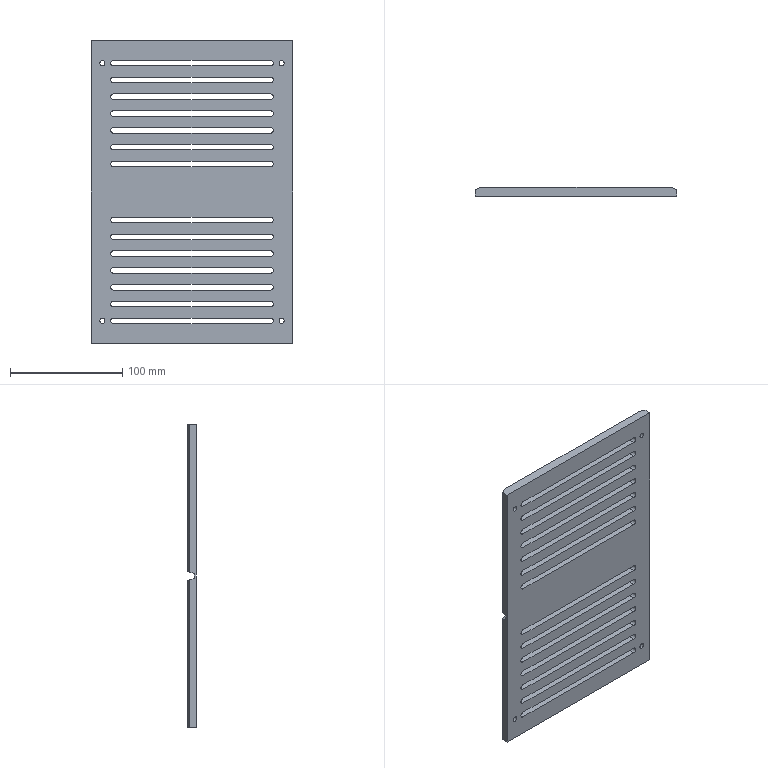Component | SolidWorks | LD101-02--Q1006-Q1-2-1 | 1 solid | 90 faces | box 180 x 8 x 270 mm | volume 297744 mm3 | plane 46 | cylinder 44 | commonest cylinder face diameters 5 x28 8 x8 4.5 x8 | material 45
build123d program:
from build123d import *

# Parameters (mm, degrees)
SKETCH1_W                                          = 180
SKETCH1_H                                          = 8
BOSS_EXTRUDE1_DEPTH                                = 135
CUT_EXTRUDE3_DEPTH                                 = 285.633
CUT_EXTRUDE4_DEPTH                                 = 226.036
CUT_EXTRUDE5_DEPTH                                 = 163.447
HOLE_SIZE_FOR_HEX_SOCKET_HEAD_CAP_SCRE_D           = 4.5
HOLE_SIZE_FOR_HEX_SOCKET_HEAD_CAP_SCRE_CBORE_D     = 8
HOLE_SIZE_FOR_HEX_SOCKET_HEAD_CAP_SCRE_CBORE_DEPTH = 4.6


with BuildPart() as part:
    # Sketch1 → Boss-Extrude1 (new, symmetric)
    with BuildSketch(Plane.XY):
        Rectangle(SKETCH1_W, SKETCH1_H)
    extrude(amount=BOSS_EXTRUDE1_DEPTH, both=True)

    # Sketch6 → Cut-Extrude3 (cut, through all)
    with BuildSketch(Plane.XY.offset(135)):
        Polygon((-90, 4), (-90, 2), (-85, 4), align=None)
        Polygon((85, 4), (90, 4), (90, 2), align=None)
    extrude(amount=-CUT_EXTRUDE3_DEPTH, mode=Mode.SUBTRACT)

    # Sketch9 → Cut-Extrude4 (cut, through all)
    with BuildSketch(Plane.ZY.offset(90)):
        Polygon((4, 4), (-4, 4), (-4.3, 4), (-1.9, -2), (1.9, -2), (4.3, 4), align=None)
    extrude(amount=-CUT_EXTRUDE4_DEPTH, mode=Mode.SUBTRACT)

    # Sketch10 → Cut-Extrude5 (cut, through all)
    with BuildSketch(Plane(origin=(0, 4, 0), x_dir=(1, 0, 0), z_dir=(0, 1, 0))):
        with BuildLine():
            Line((-70, 27.5), (70, 27.5))
            ThreePointArc((70, 27.5), (72.5, 25), (70, 22.5))
            Line((70, 22.5), (-70, 22.5))
            ThreePointArc((-70, 22.5), (-72.5, 25), (-70, 27.5))
        make_face()
        with BuildLine():
            Line((-70, 42.5), (70, 42.5))
            ThreePointArc((70, 42.5), (72.5, 40), (70, 37.5))
            Line((70, 37.5), (-70, 37.5))
            ThreePointArc((-70, 37.5), (-72.5, 40), (-70, 42.5))
        make_face()
        with BuildLine():
            Line((-70, 57.5), (70, 57.5))
            ThreePointArc((70, 57.5), (72.5, 55), (70, 52.5))
            Line((70, 52.5), (-70, 52.5))
            ThreePointArc((-70, 52.5), (-72.5, 55), (-70, 57.5))
        make_face()
        with BuildLine():
            Line((-70, 72.5), (70, 72.5))
            ThreePointArc((70, 72.5), (72.5, 70), (70, 67.5))
            Line((70, 67.5), (-70, 67.5))
            ThreePointArc((-70, 67.5), (-72.5, 70), (-70, 72.5))
        make_face()
        with BuildLine():
            Line((-70, -27.5), (70, -27.5))
            ThreePointArc((70, -27.5), (72.5, -25), (70, -22.5))
            Line((70, -22.5), (-70, -22.5))
            ThreePointArc((-70, -22.5), (-72.5, -25), (-70, -27.5))
        make_face()
        with BuildLine():
            Line((-70, -42.5), (70, -42.5))
            ThreePointArc((70, -42.5), (72.5, -40), (70, -37.5))
            Line((70, -37.5), (-70, -37.5))
            ThreePointArc((-70, -37.5), (-72.5, -40), (-70, -42.5))
        make_face()
        with BuildLine():
            Line((-70, -57.5), (70, -57.5))
            ThreePointArc((70, -57.5), (72.5, -55), (70, -52.5))
            Line((70, -52.5), (-70, -52.5))
            ThreePointArc((-70, -52.5), (-72.5, -55), (-70, -57.5))
        make_face()
        with BuildLine():
            Line((-70, -72.5), (70, -72.5))
            ThreePointArc((70, -72.5), (72.5, -70), (70, -67.5))
            Line((70, -67.5), (-70, -67.5))
            ThreePointArc((-70, -67.5), (-72.5, -70), (-70, -72.5))
        make_face()
        with BuildLine():
            Line((-70, 87.5), (70, 87.5))
            ThreePointArc((70, 87.5), (72.5, 85), (70, 82.5))
            Line((70, 82.5), (-70, 82.5))
            ThreePointArc((-70, 82.5), (-72.5, 85), (-70, 87.5))
        make_face()
        with BuildLine():
            Line((-70, 102.5), (70, 102.5))
            ThreePointArc((70, 102.5), (72.5, 100), (70, 97.5))
            Line((70, 97.5), (-70, 97.5))
            ThreePointArc((-70, 97.5), (-72.5, 100), (-70, 102.5))
        make_face()
        with BuildLine():
            Line((-70, 117.5), (70, 117.5))
            ThreePointArc((70, 117.5), (72.5, 115), (70, 112.5))
            Line((70, 112.5), (-70, 112.5))
            ThreePointArc((-70, 112.5), (-72.5, 115), (-70, 117.5))
        make_face()
        with BuildLine():
            Line((-70, -87.5), (70, -87.5))
            ThreePointArc((70, -87.5), (72.5, -85), (70, -82.5))
            Line((70, -82.5), (-70, -82.5))
            ThreePointArc((-70, -82.5), (-72.5, -85), (-70, -87.5))
        make_face()
        with BuildLine():
            Line((-70, -102.5), (70, -102.5))
            ThreePointArc((70, -102.5), (72.5, -100), (70, -97.5))
            Line((70, -97.5), (-70, -97.5))
            ThreePointArc((-70, -97.5), (-72.5, -100), (-70, -102.5))
        make_face()
        with BuildLine():
            Line((-70, -117.5), (70, -117.5))
            ThreePointArc((70, -117.5), (72.5, -115), (70, -112.5))
            Line((70, -112.5), (-70, -112.5))
            ThreePointArc((-70, -112.5), (-72.5, -115), (-70, -117.5))
        make_face()
    extrude(amount=-CUT_EXTRUDE5_DEPTH, mode=Mode.SUBTRACT)

    # Hole Size _for_ Hex Socket Head Cap Scre (through all)
    with Locations(Plane(origin=(0, 4, 0), x_dir=(1, 0, 0), z_dir=(0, 1, 0))):
        with Locations((-80, 115), (-80, -115), (80, -115), (80, 115)):
            CounterBoreHole(HOLE_SIZE_FOR_HEX_SOCKET_HEAD_CAP_SCRE_D / 2, HOLE_SIZE_FOR_HEX_SOCKET_HEAD_CAP_SCRE_CBORE_D / 2, HOLE_SIZE_FOR_HEX_SOCKET_HEAD_CAP_SCRE_CBORE_DEPTH)


solid = part.part

# Placed as in the assembly
solid = solid.moved(Location((244.21, -156.897, 146.257), (0, 0, 0)))